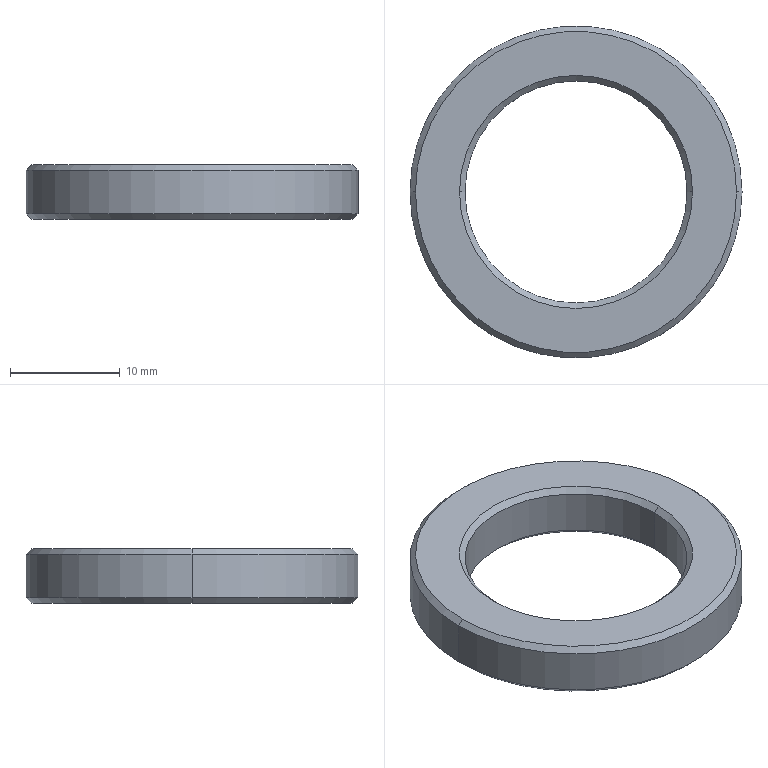Component | SolidWorks | SupportWheelAssembly-1_BearingPlate3-1 | 1 solid | 14 faces | box 30.2 x 30.2 x 5 mm | volume 1940 mm3 | cone 8 | cylinder 4 | plane 2 | commonest cylinder face diameters 20.2 x2 30.2 x2
build123d program:
from build123d import *

# Parameters (mm, degrees)
SKETCH1_R           = 15.1
SKETCH1_R_2         = 10.1
BOSS_EXTRUDE1_DEPTH = 5
CHAMFER1_SIZE       = 0.5


with BuildPart() as part:
    # Sketch1 → Boss-Extrude1 (new body)
    with BuildSketch(Plane.XY):
        Circle(SKETCH1_R)
        Circle(SKETCH1_R_2, mode=Mode.SUBTRACT)
    extrude(amount=BOSS_EXTRUDE1_DEPTH)

    # Chamfer1
    chamfer1_edges = [part.edges().sort_by_distance(p)[0] for p in [
        (-15.1, 0, 0),
        (-15.1, 0, 5),
        (-10.1, 0, 0),
        (-10.1, 0, 5),
    ]]
    chamfer(chamfer1_edges, length=CHAMFER1_SIZE)


solid = part.part

# Placed as in the assembly
solid = solid.moved(Location((-187.007, -195.411, 515), (0, 0, 0)))
STEP:
#1=CARTESIAN_POINT('',(-7.76,-7.693,20.453));
#2=VERTEX_POINT('',#1);
#3=CARTESIAN_POINT('',(-6.965,-7.693,20.453));
#4=VERTEX_POINT('',#3);
#5=CARTESIAN_POINT('',(-7.362,-7.693,20.453));
#6=DIRECTION('',(0.,0.,1.));
#7=DIRECTION('',(1.,0.,0.));
#8=AXIS2_PLACEMENT_3D('',#5,#6,#7);
#9=CIRCLE('',#8,0.3976);
#10=EDGE_CURVE('',#2,#4,#9,.T.);
#11=ORIENTED_EDGE('',*,*,#10,.F.);
#12=CARTESIAN_POINT('',(-7.78,-7.693,20.472));
#13=VERTEX_POINT('',#12);
#14=CARTESIAN_POINT('',(-7.76,-7.693,20.453));
#15=DIRECTION('',(-0.7071,0.,0.7071));
#16=VECTOR('',#15,39.37);
#17=LINE('',#14,#16);
#18=EDGE_CURVE('',#2,#13,#17,.T.);
#19=ORIENTED_EDGE('',*,*,#18,.T.);
#20=CARTESIAN_POINT('',(-6.945,-7.693,20.472));
#21=VERTEX_POINT('',#20);
#22=CARTESIAN_POINT('',(-7.362,-7.693,20.472));
#23=DIRECTION('',(0.,0.,-1.));
#24=DIRECTION('',(1.,0.,0.));
#25=AXIS2_PLACEMENT_3D('',#22,#23,#24);
#26=CIRCLE('',#25,0.4173);
#27=EDGE_CURVE('',#21,#13,#26,.T.);
#28=ORIENTED_EDGE('',*,*,#27,.F.);
#29=CARTESIAN_POINT('',(-6.965,-7.693,20.453));
#30=DIRECTION('',(0.7071,0.,0.7071));
#31=VECTOR('',#30,39.37);
#32=LINE('',#29,#31);
#33=EDGE_CURVE('',#4,#21,#32,.T.);
#34=ORIENTED_EDGE('',*,*,#33,.F.);
#35=EDGE_LOOP('',(#11,#19,#28,#34));
#36=FACE_OUTER_BOUND('',#35,.T.);
#37=CARTESIAN_POINT('',(-7.362,-7.693,20.453));
#38=DIRECTION('',(0.,0.,1.));
#39=DIRECTION('',(1.,0.,0.));
#40=AXIS2_PLACEMENT_3D('',#37,#38,#39);
#41=CONICAL_SURFACE('',#40,0.3976,0.7854);
#42=ADVANCED_FACE('',(#36),#41,.F.);
#43=CARTESIAN_POINT('',(-6.965,-7.693,20.295));
#44=VERTEX_POINT('',#43);
#45=CARTESIAN_POINT('',(-7.76,-7.693,20.295));
#46=VERTEX_POINT('',#45);
#47=CARTESIAN_POINT('',(-7.362,-7.693,20.295));
#48=DIRECTION('',(0.,0.,-1.));
#49=DIRECTION('',(1.,0.,0.));
#50=AXIS2_PLACEMENT_3D('',#47,#48,#49);
#51=CIRCLE('',#50,0.3976);
#52=EDGE_CURVE('',#44,#46,#51,.T.);
#53=ORIENTED_EDGE('',*,*,#52,.F.);
#54=CARTESIAN_POINT('',(-6.945,-7.693,20.276));
#55=VERTEX_POINT('',#54);
#56=CARTESIAN_POINT('',(-6.945,-7.693,20.276));
#57=DIRECTION('',(0.7071,0.,-0.7071));
#58=VECTOR('',#57,39.37);
#59=LINE('',#56,#58);
#60=EDGE_CURVE('',#44,#55,#59,.T.);
#61=ORIENTED_EDGE('',*,*,#60,.T.);
#62=CARTESIAN_POINT('',(-7.78,-7.693,20.276));
#63=VERTEX_POINT('',#62);
#64=CARTESIAN_POINT('',(-7.362,-7.693,20.276));
#65=DIRECTION('',(0.,0.,1.));
#66=DIRECTION('',(1.,0.,0.));
#67=AXIS2_PLACEMENT_3D('',#64,#65,#66);
#68=CIRCLE('',#67,0.4173);
#69=EDGE_CURVE('',#63,#55,#68,.T.);
#70=ORIENTED_EDGE('',*,*,#69,.F.);
#71=CARTESIAN_POINT('',(-7.78,-7.693,20.276));
#72=DIRECTION('',(-0.7071,0.,-0.7071));
#73=VECTOR('',#72,39.37);
#74=LINE('',#71,#73);
#75=EDGE_CURVE('',#46,#63,#74,.T.);
#76=ORIENTED_EDGE('',*,*,#75,.F.);
#77=EDGE_LOOP('',(#53,#61,#70,#76));
#78=FACE_OUTER_BOUND('',#77,.T.);
#79=CARTESIAN_POINT('',(-7.362,-7.693,20.276));
#80=DIRECTION('',(0.,0.,-1.));
#81=DIRECTION('',(-1.,0.,0.));
#82=AXIS2_PLACEMENT_3D('',#79,#80,#81);
#83=CONICAL_SURFACE('',#82,0.4173,0.7854);
#84=ADVANCED_FACE('',(#78),#83,.F.);
#85=CARTESIAN_POINT('',(-6.788,-7.693,20.472));
#86=VERTEX_POINT('',#85);
#87=CARTESIAN_POINT('',(-7.937,-7.693,20.472));
#88=VERTEX_POINT('',#87);
#89=CARTESIAN_POINT('',(-7.362,-7.693,20.472));
#90=DIRECTION('',(0.,0.,1.));
#91=DIRECTION('',(1.,0.,0.));
#92=AXIS2_PLACEMENT_3D('',#89,#90,#91);
#93=CIRCLE('',#92,0.5748);
#94=EDGE_CURVE('',#86,#88,#93,.T.);
#95=ORIENTED_EDGE('',*,*,#94,.F.);
#96=CARTESIAN_POINT('',(-6.768,-7.693,20.453));
#97=VERTEX_POINT('',#96);
#98=CARTESIAN_POINT('',(-6.788,-7.693,20.472));
#99=DIRECTION('',(0.7071,0.,-0.7071));
#100=VECTOR('',#99,39.37);
#101=LINE('',#98,#100);
#102=EDGE_CURVE('',#86,#97,#101,.T.);
#103=ORIENTED_EDGE('',*,*,#102,.T.);
#104=CARTESIAN_POINT('',(-7.957,-7.693,20.453));
#105=VERTEX_POINT('',#104);
#106=CARTESIAN_POINT('',(-7.362,-7.693,20.453));
#107=DIRECTION('',(0.,0.,-1.));
#108=DIRECTION('',(1.,0.,0.));
#109=AXIS2_PLACEMENT_3D('',#106,#107,#108);
#110=CIRCLE('',#109,0.5945);
#111=EDGE_CURVE('',#105,#97,#110,.T.);
#112=ORIENTED_EDGE('',*,*,#111,.F.);
#113=CARTESIAN_POINT('',(-7.937,-7.693,20.472));
#114=DIRECTION('',(-0.7071,0.,-0.7071));
#115=VECTOR('',#114,39.37);
#116=LINE('',#113,#115);
#117=EDGE_CURVE('',#88,#105,#116,.T.);
#118=ORIENTED_EDGE('',*,*,#117,.F.);
#119=EDGE_LOOP('',(#95,#103,#112,#118));
#120=FACE_OUTER_BOUND('',#119,.T.);
#121=CARTESIAN_POINT('',(-7.362,-7.693,20.472));
#122=DIRECTION('',(0.,0.,-1.));
#123=DIRECTION('',(-1.,0.,0.));
#124=AXIS2_PLACEMENT_3D('',#121,#122,#123);
#125=CONICAL_SURFACE('',#124,0.5748,0.7854);
#126=ADVANCED_FACE('',(#120),#125,.T.);
#127=CARTESIAN_POINT('',(-7.937,-7.693,20.276));
#128=VERTEX_POINT('',#127);
#129=CARTESIAN_POINT('',(-6.788,-7.693,20.276));
#130=VERTEX_POINT('',#129);
#131=CARTESIAN_POINT('',(-7.362,-7.693,20.276));
#132=DIRECTION('',(0.,0.,-1.));
#133=DIRECTION('',(1.,0.,0.));
#134=AXIS2_PLACEMENT_3D('',#131,#132,#133);
#135=CIRCLE('',#134,0.5748);
#136=EDGE_CURVE('',#128,#130,#135,.T.);
#137=ORIENTED_EDGE('',*,*,#136,.F.);
#138=CARTESIAN_POINT('',(-7.957,-7.693,20.295));
#139=VERTEX_POINT('',#138);
#140=CARTESIAN_POINT('',(-7.957,-7.693,20.295));
#141=DIRECTION('',(-0.7071,0.,0.7071));
#142=VECTOR('',#141,39.37);
#143=LINE('',#140,#142);
#144=EDGE_CURVE('',#128,#139,#143,.T.);
#145=ORIENTED_EDGE('',*,*,#144,.T.);
#146=CARTESIAN_POINT('',(-6.768,-7.693,20.295));
#147=VERTEX_POINT('',#146);
#148=CARTESIAN_POINT('',(-7.362,-7.693,20.295));
#149=DIRECTION('',(0.,0.,1.));
#150=DIRECTION('',(1.,0.,0.));
#151=AXIS2_PLACEMENT_3D('',#148,#149,#150);
#152=CIRCLE('',#151,0.5945);
#153=EDGE_CURVE('',#147,#139,#152,.T.);
#154=ORIENTED_EDGE('',*,*,#153,.F.);
#155=CARTESIAN_POINT('',(-6.768,-7.693,20.295));
#156=DIRECTION('',(0.7071,0.,0.7071));
#157=VECTOR('',#156,39.37);
#158=LINE('',#155,#157);
#159=EDGE_CURVE('',#130,#147,#158,.T.);
#160=ORIENTED_EDGE('',*,*,#159,.F.);
#161=EDGE_LOOP('',(#137,#145,#154,#160));
#162=FACE_OUTER_BOUND('',#161,.T.);
#163=CARTESIAN_POINT('',(-7.362,-7.693,20.295));
#164=DIRECTION('',(0.,0.,1.));
#165=DIRECTION('',(1.,0.,0.));
#166=AXIS2_PLACEMENT_3D('',#163,#164,#165);
#167=CONICAL_SURFACE('',#166,0.5945,0.7854);
#168=ADVANCED_FACE('',(#162),#167,.T.);
#169=ORIENTED_EDGE('',*,*,#10,.T.);
#170=CARTESIAN_POINT('',(-6.965,-7.693,20.472));
#171=DIRECTION('',(0.,0.,-1.));
#172=VECTOR('',#171,39.37);
#173=LINE('',#170,#172);
#174=EDGE_CURVE('',#4,#44,#173,.T.);
#175=ORIENTED_EDGE('',*,*,#174,.T.);
#176=ORIENTED_EDGE('',*,*,#52,.T.);
#177=CARTESIAN_POINT('',(-7.76,-7.693,20.472));
#178=DIRECTION('',(0.,0.,-1.));
#179=VECTOR('',#178,39.37);
#180=LINE('',#177,#179);
#181=EDGE_CURVE('',#2,#46,#180,.T.);
#182=ORIENTED_EDGE('',*,*,#181,.F.);
#183=EDGE_LOOP('',(#169,#175,#176,#182));
#184=FACE_OUTER_BOUND('',#183,.T.);
#185=CARTESIAN_POINT('',(-7.362,-7.693,20.472));
#186=DIRECTION('',(0.,0.,-1.));
#187=DIRECTION('',(-1.,0.,0.));
#188=AXIS2_PLACEMENT_3D('',#185,#186,#187);
#189=CYLINDRICAL_SURFACE('',#188,0.3976);
#190=ADVANCED_FACE('',(#184),#189,.F.);
#191=ORIENTED_EDGE('',*,*,#111,.T.);
#192=CARTESIAN_POINT('',(-6.768,-7.693,20.472));
#193=DIRECTION('',(0.,0.,-1.));
#194=VECTOR('',#193,39.37);
#195=LINE('',#192,#194);
#196=EDGE_CURVE('',#97,#147,#195,.T.);
#197=ORIENTED_EDGE('',*,*,#196,.T.);
#198=ORIENTED_EDGE('',*,*,#153,.T.);
#199=CARTESIAN_POINT('',(-7.957,-7.693,20.472));
#200=DIRECTION('',(0.,0.,-1.));
#201=VECTOR('',#200,39.37);
#202=LINE('',#199,#201);
#203=EDGE_CURVE('',#105,#139,#202,.T.);
#204=ORIENTED_EDGE('',*,*,#203,.F.);
#205=EDGE_LOOP('',(#191,#197,#198,#204));
#206=FACE_OUTER_BOUND('',#205,.T.);
#207=CARTESIAN_POINT('',(-7.362,-7.693,20.472));
#208=DIRECTION('',(0.,0.,-1.));
#209=DIRECTION('',(-1.,0.,0.));
#210=AXIS2_PLACEMENT_3D('',#207,#208,#209);
#211=CYLINDRICAL_SURFACE('',#210,0.5945);
#212=ADVANCED_FACE('',(#206),#211,.T.);
#213=CARTESIAN_POINT('',(-7.362,-7.693,20.472));
#214=DIRECTION('',(0.,0.,1.));
#215=DIRECTION('',(1.,0.,0.));
#216=AXIS2_PLACEMENT_3D('',#213,#214,#215);
#217=CIRCLE('',#216,0.5748);
#218=EDGE_CURVE('',#88,#86,#217,.T.);
#219=ORIENTED_EDGE('',*,*,#218,.T.);
#220=ORIENTED_EDGE('',*,*,#94,.T.);
#221=EDGE_LOOP('',(#219,#220));
#222=FACE_OUTER_BOUND('',#221,.T.);
#223=ORIENTED_EDGE('',*,*,#27,.T.);
#224=CARTESIAN_POINT('',(-7.362,-7.693,20.472));
#225=DIRECTION('',(0.,0.,-1.));
#226=DIRECTION('',(1.,0.,0.));
#227=AXIS2_PLACEMENT_3D('',#224,#225,#226);
#228=CIRCLE('',#227,0.4173);
#229=EDGE_CURVE('',#13,#21,#228,.T.);
#230=ORIENTED_EDGE('',*,*,#229,.T.);
#231=EDGE_LOOP('',(#223,#230));
#232=FACE_BOUND('',#231,.T.);
#233=CARTESIAN_POINT('',(-7.362,-7.693,20.472));
#234=DIRECTION('',(0.,0.,1.));
#235=DIRECTION('',(1.,0.,0.));
#236=AXIS2_PLACEMENT_3D('',#233,#234,#235);
#237=PLANE('',#236);
#238=ADVANCED_FACE('',(#222,#232),#237,.T.);
#239=CARTESIAN_POINT('',(-7.362,-7.693,20.276));
#240=DIRECTION('',(0.,0.,-1.));
#241=DIRECTION('',(1.,0.,0.));
#242=AXIS2_PLACEMENT_3D('',#239,#240,#241);
#243=CIRCLE('',#242,0.5748);
#244=EDGE_CURVE('',#130,#128,#243,.T.);
#245=ORIENTED_EDGE('',*,*,#244,.T.);
#246=ORIENTED_EDGE('',*,*,#136,.T.);
#247=EDGE_LOOP('',(#245,#246));
#248=FACE_OUTER_BOUND('',#247,.T.);
#249=ORIENTED_EDGE('',*,*,#69,.T.);
#250=CARTESIAN_POINT('',(-7.362,-7.693,20.276));
#251=DIRECTION('',(0.,0.,1.));
#252=DIRECTION('',(1.,0.,0.));
#253=AXIS2_PLACEMENT_3D('',#250,#251,#252);
#254=CIRCLE('',#253,0.4173);
#255=EDGE_CURVE('',#55,#63,#254,.T.);
#256=ORIENTED_EDGE('',*,*,#255,.T.);
#257=EDGE_LOOP('',(#249,#256));
#258=FACE_BOUND('',#257,.T.);
#259=CARTESIAN_POINT('',(-7.362,-7.693,20.276));
#260=DIRECTION('',(0.,0.,1.));
#261=DIRECTION('',(1.,0.,0.));
#262=AXIS2_PLACEMENT_3D('',#259,#260,#261);
#263=PLANE('',#262);
#264=ADVANCED_FACE('',(#248,#258),#263,.F.);
#265=ORIENTED_EDGE('',*,*,#196,.F.);
#266=CARTESIAN_POINT('',(-7.362,-7.693,20.453));
#267=DIRECTION('',(0.,0.,-1.));
#268=DIRECTION('',(1.,0.,0.));
#269=AXIS2_PLACEMENT_3D('',#266,#267,#268);
#270=CIRCLE('',#269,0.5945);
#271=EDGE_CURVE('',#97,#105,#270,.T.);
#272=ORIENTED_EDGE('',*,*,#271,.T.);
#273=ORIENTED_EDGE('',*,*,#203,.T.);
#274=CARTESIAN_POINT('',(-7.362,-7.693,20.295));
#275=DIRECTION('',(0.,0.,1.));
#276=DIRECTION('',(1.,0.,0.));
#277=AXIS2_PLACEMENT_3D('',#274,#275,#276);
#278=CIRCLE('',#277,0.5945);
#279=EDGE_CURVE('',#139,#147,#278,.T.);
#280=ORIENTED_EDGE('',*,*,#279,.T.);
#281=EDGE_LOOP('',(#265,#272,#273,#280));
#282=FACE_OUTER_BOUND('',#281,.T.);
#283=CARTESIAN_POINT('',(-7.362,-7.693,20.472));
#284=DIRECTION('',(0.,0.,-1.));
#285=DIRECTION('',(-1.,0.,0.));
#286=AXIS2_PLACEMENT_3D('',#283,#284,#285);
#287=CYLINDRICAL_SURFACE('',#286,0.5945);
#288=ADVANCED_FACE('',(#282),#287,.T.);
#289=ORIENTED_EDGE('',*,*,#174,.F.);
#290=CARTESIAN_POINT('',(-7.362,-7.693,20.453));
#291=DIRECTION('',(0.,0.,1.));
#292=DIRECTION('',(1.,0.,0.));
#293=AXIS2_PLACEMENT_3D('',#290,#291,#292);
#294=CIRCLE('',#293,0.3976);
#295=EDGE_CURVE('',#4,#2,#294,.T.);
#296=ORIENTED_EDGE('',*,*,#295,.T.);
#297=ORIENTED_EDGE('',*,*,#181,.T.);
#298=CARTESIAN_POINT('',(-7.362,-7.693,20.295));
#299=DIRECTION('',(0.,0.,-1.));
#300=DIRECTION('',(1.,0.,0.));
#301=AXIS2_PLACEMENT_3D('',#298,#299,#300);
#302=CIRCLE('',#301,0.3976);
#303=EDGE_CURVE('',#46,#44,#302,.T.);
#304=ORIENTED_EDGE('',*,*,#303,.T.);
#305=EDGE_LOOP('',(#289,#296,#297,#304));
#306=FACE_OUTER_BOUND('',#305,.T.);
#307=CARTESIAN_POINT('',(-7.362,-7.693,20.472));
#308=DIRECTION('',(0.,0.,-1.));
#309=DIRECTION('',(-1.,0.,0.));
#310=AXIS2_PLACEMENT_3D('',#307,#308,#309);
#311=CYLINDRICAL_SURFACE('',#310,0.3976);
#312=ADVANCED_FACE('',(#306),#311,.F.);
#313=ORIENTED_EDGE('',*,*,#144,.F.);
#314=ORIENTED_EDGE('',*,*,#244,.F.);
#315=ORIENTED_EDGE('',*,*,#159,.T.);
#316=ORIENTED_EDGE('',*,*,#279,.F.);
#317=EDGE_LOOP('',(#313,#314,#315,#316));
#318=FACE_OUTER_BOUND('',#317,.T.);
#319=CARTESIAN_POINT('',(-7.362,-7.693,20.295));
#320=DIRECTION('',(0.,0.,1.));
#321=DIRECTION('',(1.,0.,0.));
#322=AXIS2_PLACEMENT_3D('',#319,#320,#321);
#323=CONICAL_SURFACE('',#322,0.5945,0.7854);
#324=ADVANCED_FACE('',(#318),#323,.T.);
#325=ORIENTED_EDGE('',*,*,#102,.F.);
#326=ORIENTED_EDGE('',*,*,#218,.F.);
#327=ORIENTED_EDGE('',*,*,#117,.T.);
#328=ORIENTED_EDGE('',*,*,#271,.F.);
#329=EDGE_LOOP('',(#325,#326,#327,#328));
#330=FACE_OUTER_BOUND('',#329,.T.);
#331=CARTESIAN_POINT('',(-7.362,-7.693,20.472));
#332=DIRECTION('',(0.,0.,-1.));
#333=DIRECTION('',(-1.,0.,0.));
#334=AXIS2_PLACEMENT_3D('',#331,#332,#333);
#335=CONICAL_SURFACE('',#334,0.5748,0.7854);
#336=ADVANCED_FACE('',(#330),#335,.T.);
#337=ORIENTED_EDGE('',*,*,#60,.F.);
#338=ORIENTED_EDGE('',*,*,#303,.F.);
#339=ORIENTED_EDGE('',*,*,#75,.T.);
#340=ORIENTED_EDGE('',*,*,#255,.F.);
#341=EDGE_LOOP('',(#337,#338,#339,#340));
#342=FACE_OUTER_BOUND('',#341,.T.);
#343=CARTESIAN_POINT('',(-7.362,-7.693,20.276));
#344=DIRECTION('',(0.,0.,-1.));
#345=DIRECTION('',(-1.,0.,0.));
#346=AXIS2_PLACEMENT_3D('',#343,#344,#345);
#347=CONICAL_SURFACE('',#346,0.4173,0.7854);
#348=ADVANCED_FACE('',(#342),#347,.F.);
#349=ORIENTED_EDGE('',*,*,#18,.F.);
#350=ORIENTED_EDGE('',*,*,#295,.F.);
#351=ORIENTED_EDGE('',*,*,#33,.T.);
#352=ORIENTED_EDGE('',*,*,#229,.F.);
#353=EDGE_LOOP('',(#349,#350,#351,#352));
#354=FACE_OUTER_BOUND('',#353,.T.);
#355=CARTESIAN_POINT('',(-7.362,-7.693,20.453));
#356=DIRECTION('',(0.,0.,1.));
#357=DIRECTION('',(1.,0.,0.));
#358=AXIS2_PLACEMENT_3D('',#355,#356,#357);
#359=CONICAL_SURFACE('',#358,0.3976,0.7854);
#360=ADVANCED_FACE('',(#354),#359,.F.);
#361=CLOSED_SHELL('',(#42,#84,#126,#168,#190,#212,#238,#264,#288,#312,#324,#336,#348,#360));
#362=MANIFOLD_SOLID_BREP('',#361);
#363=CARTESIAN_POINT('',(0.,0.,0.));
#364=DIRECTION('',(0.,0.,1.));
#365=DIRECTION('',(1.,0.,0.));
#366=AXIS2_PLACEMENT_3D('',#363,#364,#365);
#367=(LENGTH_UNIT()NAMED_UNIT(*)SI_UNIT($,.METRE.));
#368=LENGTH_MEASURE_WITH_UNIT(LENGTH_MEASURE(0.0254),#367);
#369=DIMENSIONAL_EXPONENTS(1.,0.,0.,0.,0.,0.,0.);
#370=(CONVERSION_BASED_UNIT('',#368)LENGTH_UNIT()NAMED_UNIT(#369));
#371=UNCERTAINTY_MEASURE_WITH_UNIT(LENGTH_MEASURE(0.00001),#370,'','');
#372=(NAMED_UNIT(*)PLANE_ANGLE_UNIT()SI_UNIT($,.RADIAN.));
#373=(NAMED_UNIT(*)SI_UNIT($,.STERADIAN.)SOLID_ANGLE_UNIT());
#374=(GEOMETRIC_REPRESENTATION_CONTEXT(3)GLOBAL_UNCERTAINTY_ASSIGNED_CONTEXT((#371))GLOBAL_UNIT_ASSIGNED_CONTEXT((#370,#372,#373))REPRESENTATION_CONTEXT('',''));
#375=ADVANCED_BREP_SHAPE_REPRESENTATION('',(#362,#366),#374);
#376=COLOUR_RGB('',0.7922,0.8196,0.9333);
#377=FILL_AREA_STYLE_COLOUR('',#376);
#378=FILL_AREA_STYLE('',(#377));
#379=SURFACE_STYLE_FILL_AREA(#378);
#380=SURFACE_SIDE_STYLE('',(#379));
#381=SURFACE_STYLE_USAGE(.BOTH.,#380);
#382=PRESENTATION_STYLE_ASSIGNMENT((#381));
#383=STYLED_ITEM('',(#382),#362);
#384=PRESENTATION_LAYER_ASSIGNMENT('','',(#383));
#385=(LENGTH_UNIT()NAMED_UNIT(*)SI_UNIT($,.METRE.));
#386=LENGTH_MEASURE_WITH_UNIT(LENGTH_MEASURE(0.0254),#385);
#387=DIMENSIONAL_EXPONENTS(1.,0.,0.,0.,0.,0.,0.);
#388=(CONVERSION_BASED_UNIT('',#386)LENGTH_UNIT()NAMED_UNIT(#387));
#389=UNCERTAINTY_MEASURE_WITH_UNIT(LENGTH_MEASURE(0.00001),#388,'','');
#390=(NAMED_UNIT(*)PLANE_ANGLE_UNIT()SI_UNIT($,.RADIAN.));
#391=(NAMED_UNIT(*)SI_UNIT($,.STERADIAN.)SOLID_ANGLE_UNIT());
#392=(GEOMETRIC_REPRESENTATION_CONTEXT(3)GLOBAL_UNCERTAINTY_ASSIGNED_CONTEXT((#389))GLOBAL_UNIT_ASSIGNED_CONTEXT((#388,#390,#391))REPRESENTATION_CONTEXT('',''));
#393=MECHANICAL_DESIGN_GEOMETRIC_PRESENTATION_REPRESENTATION('',(#383),#392);